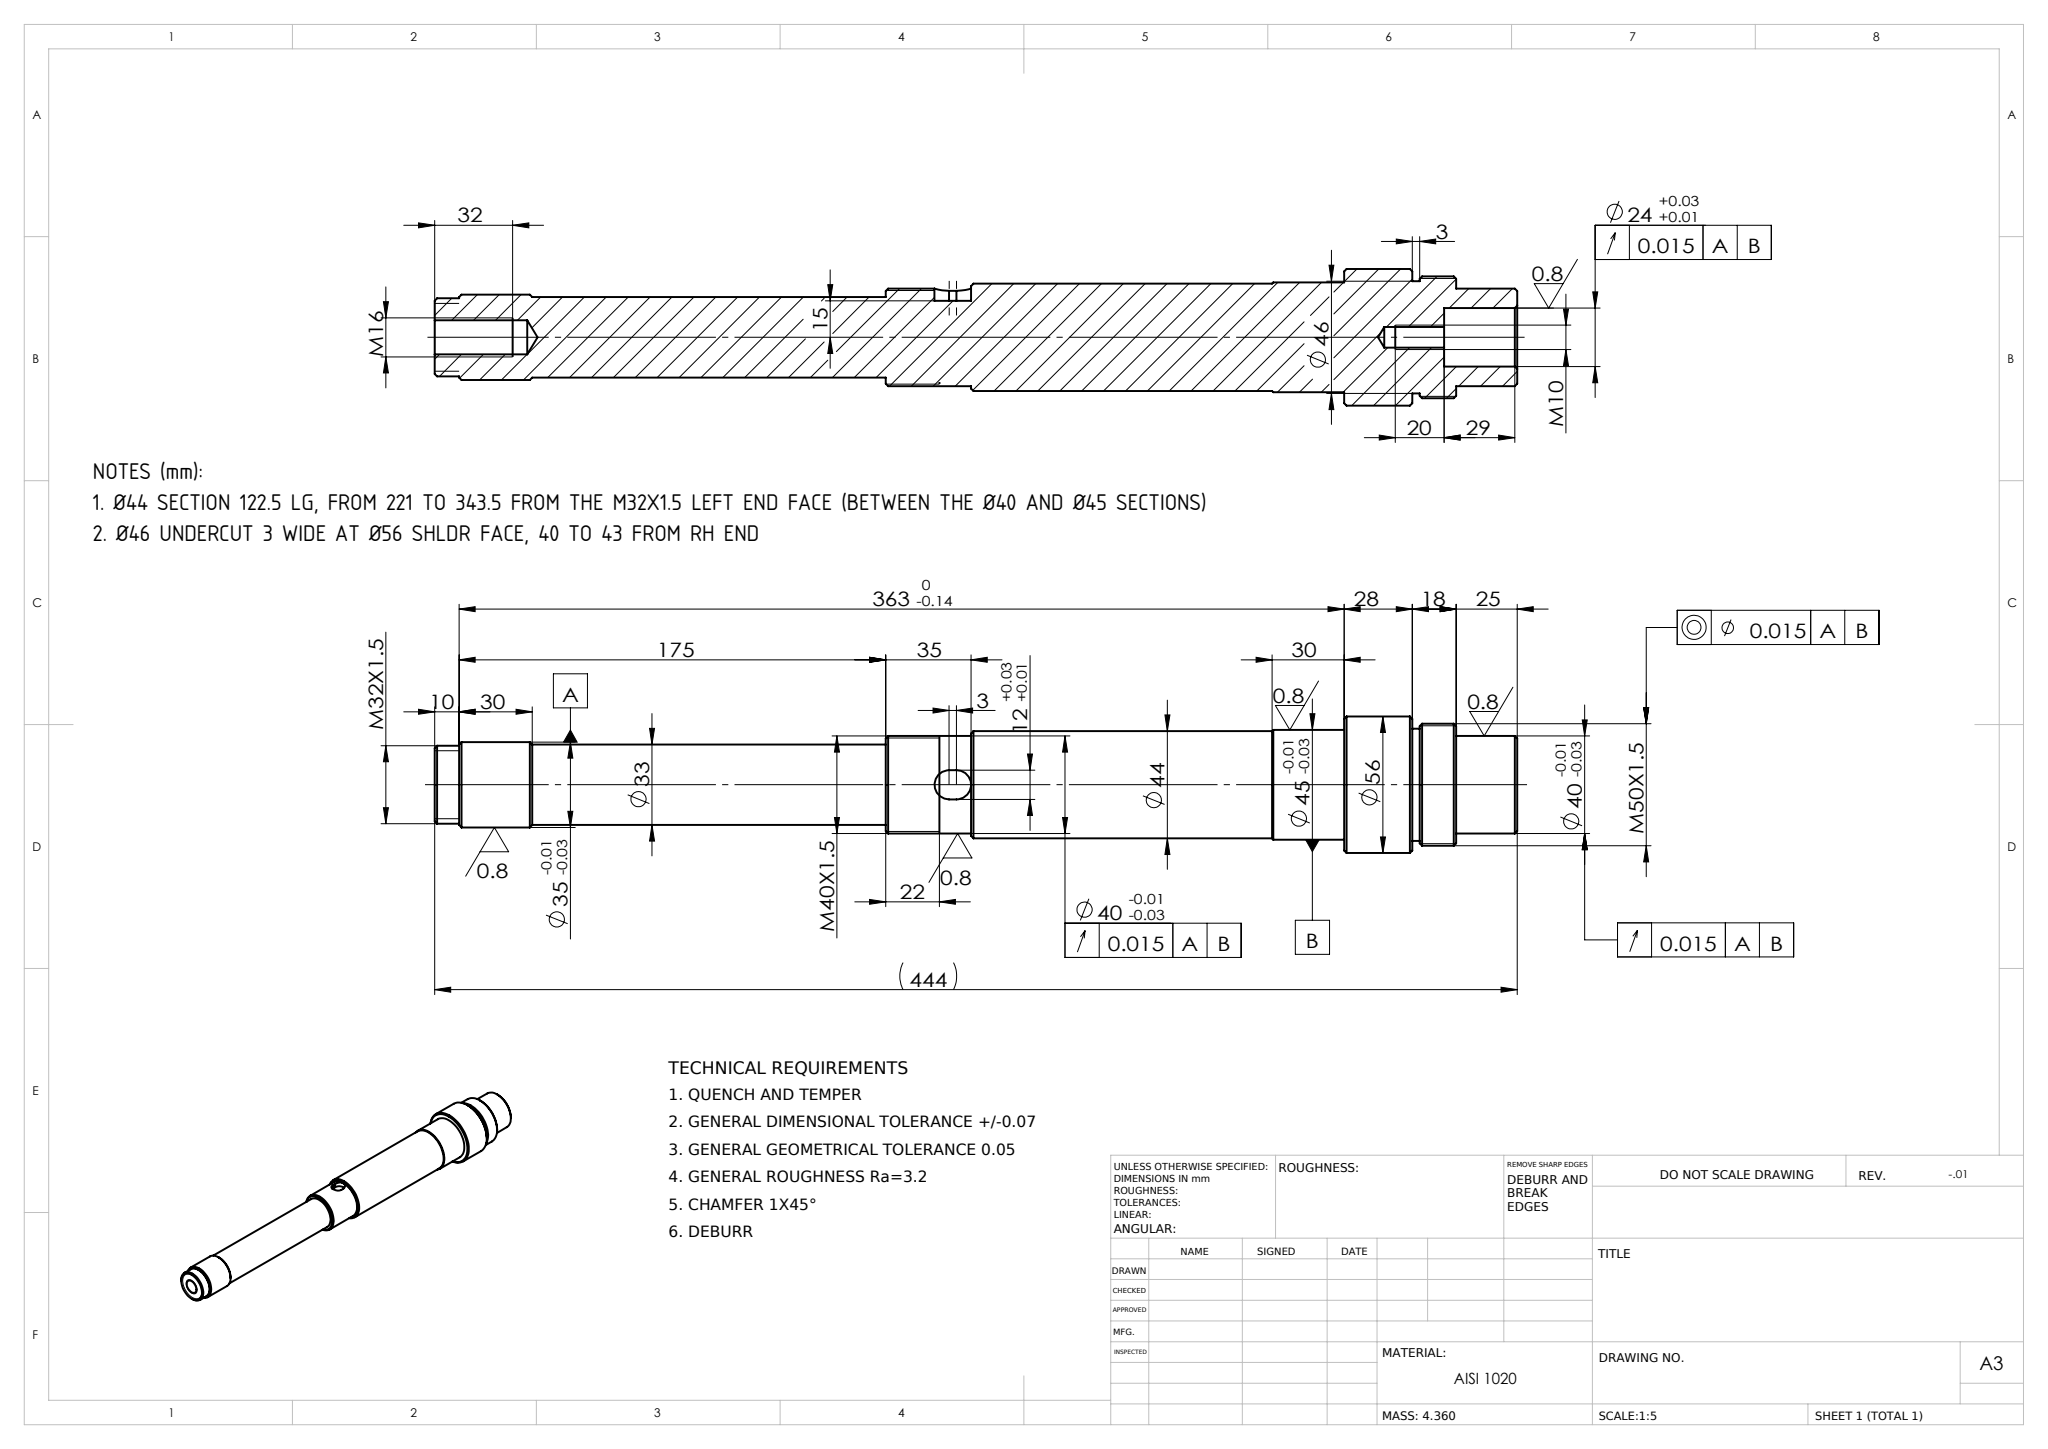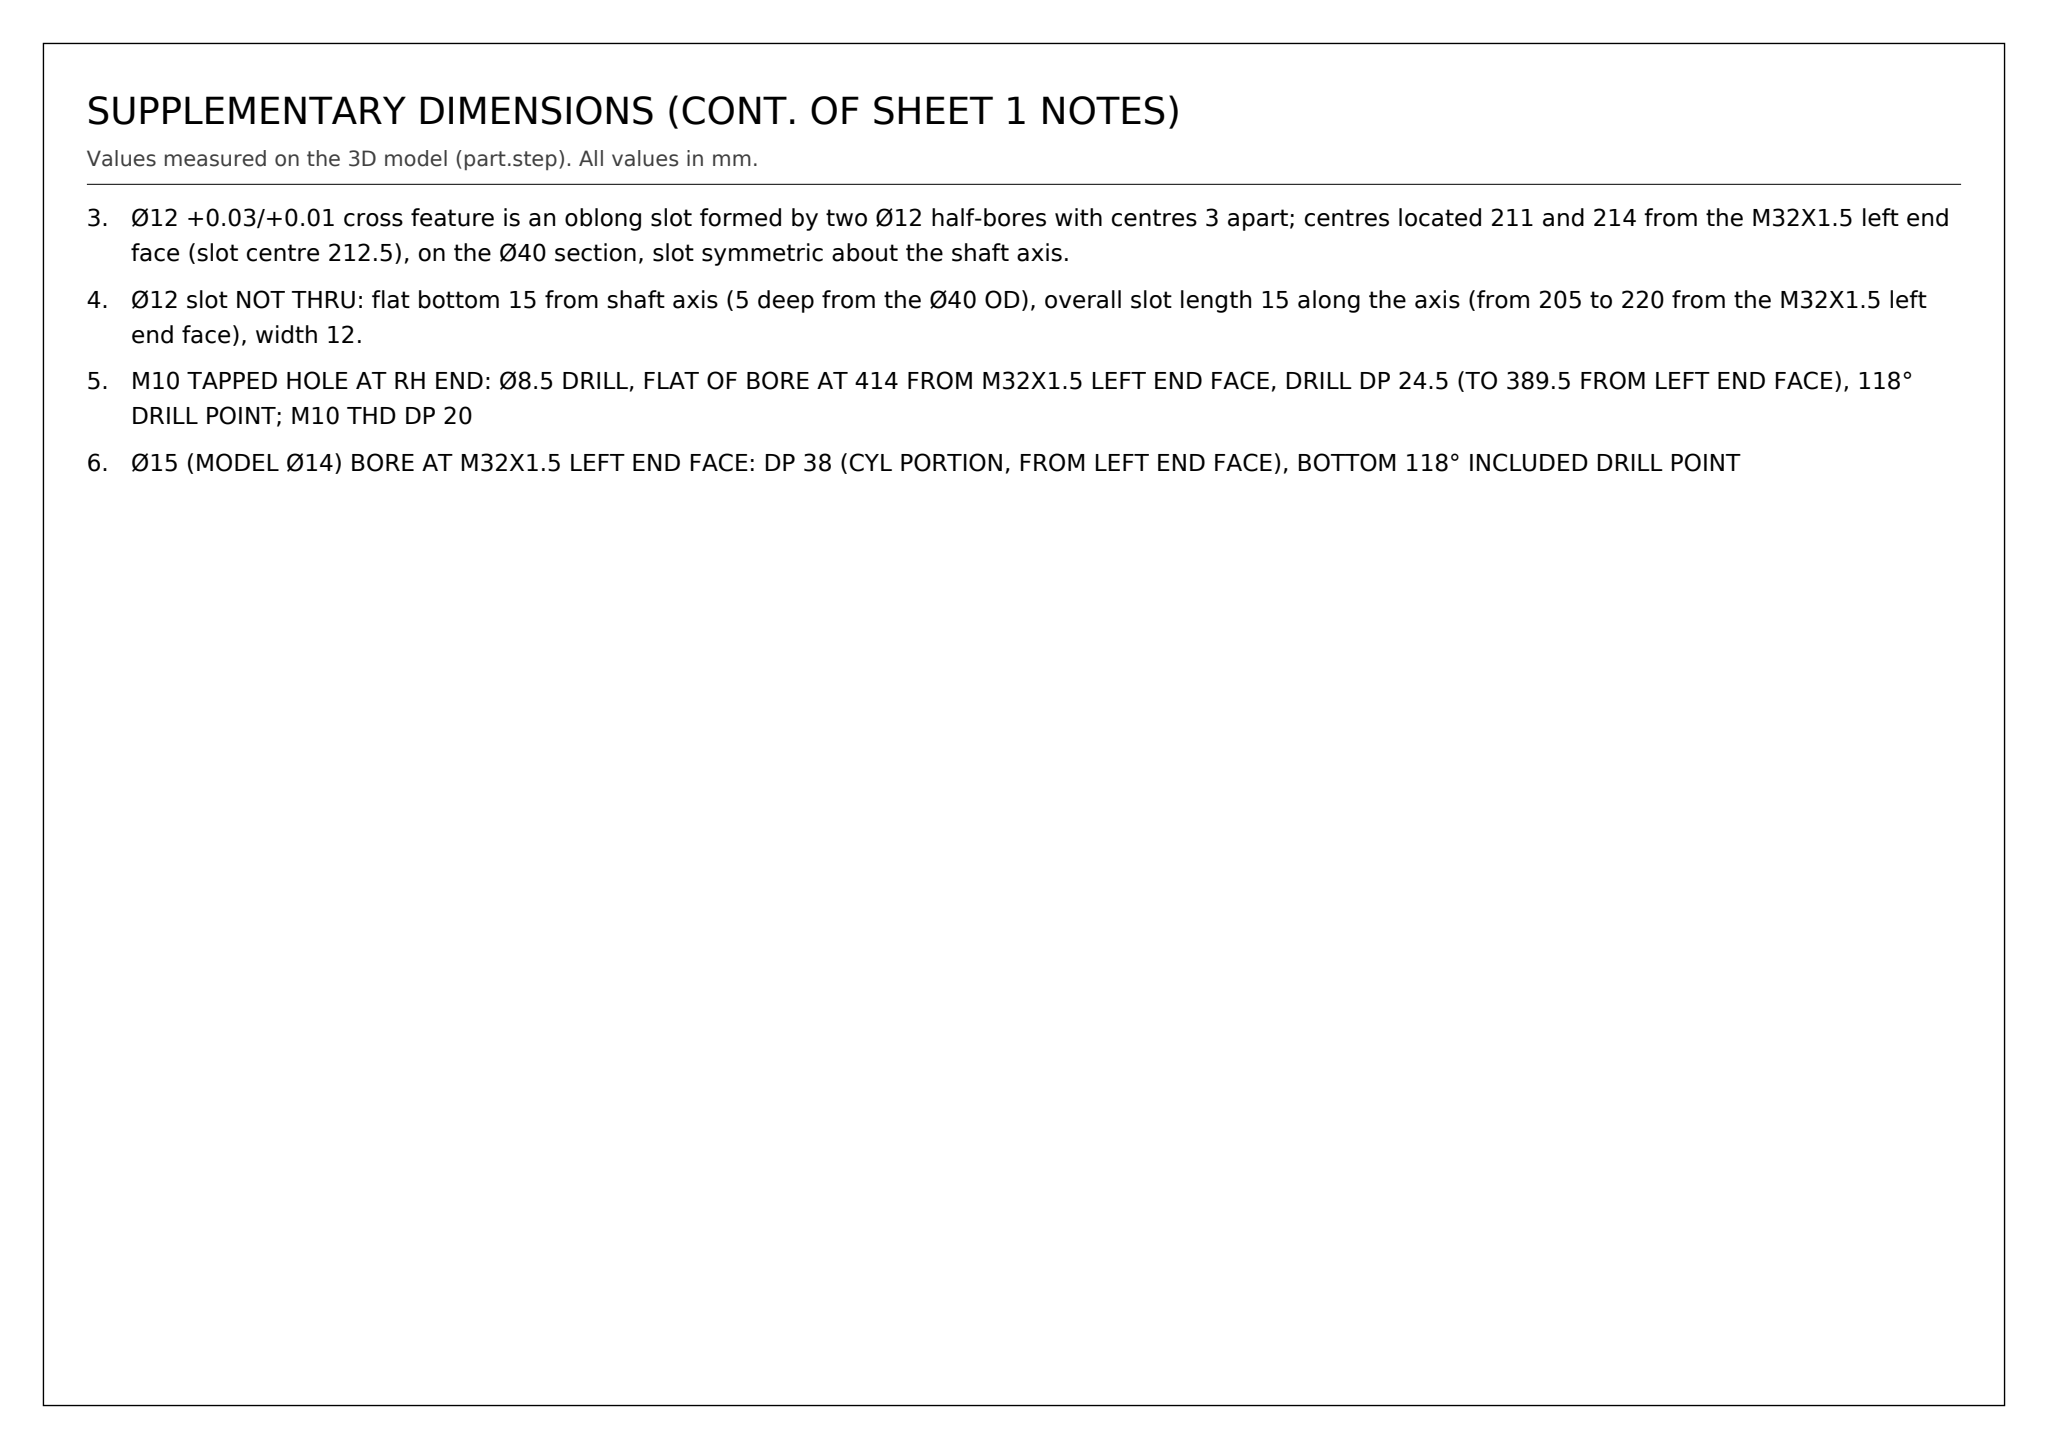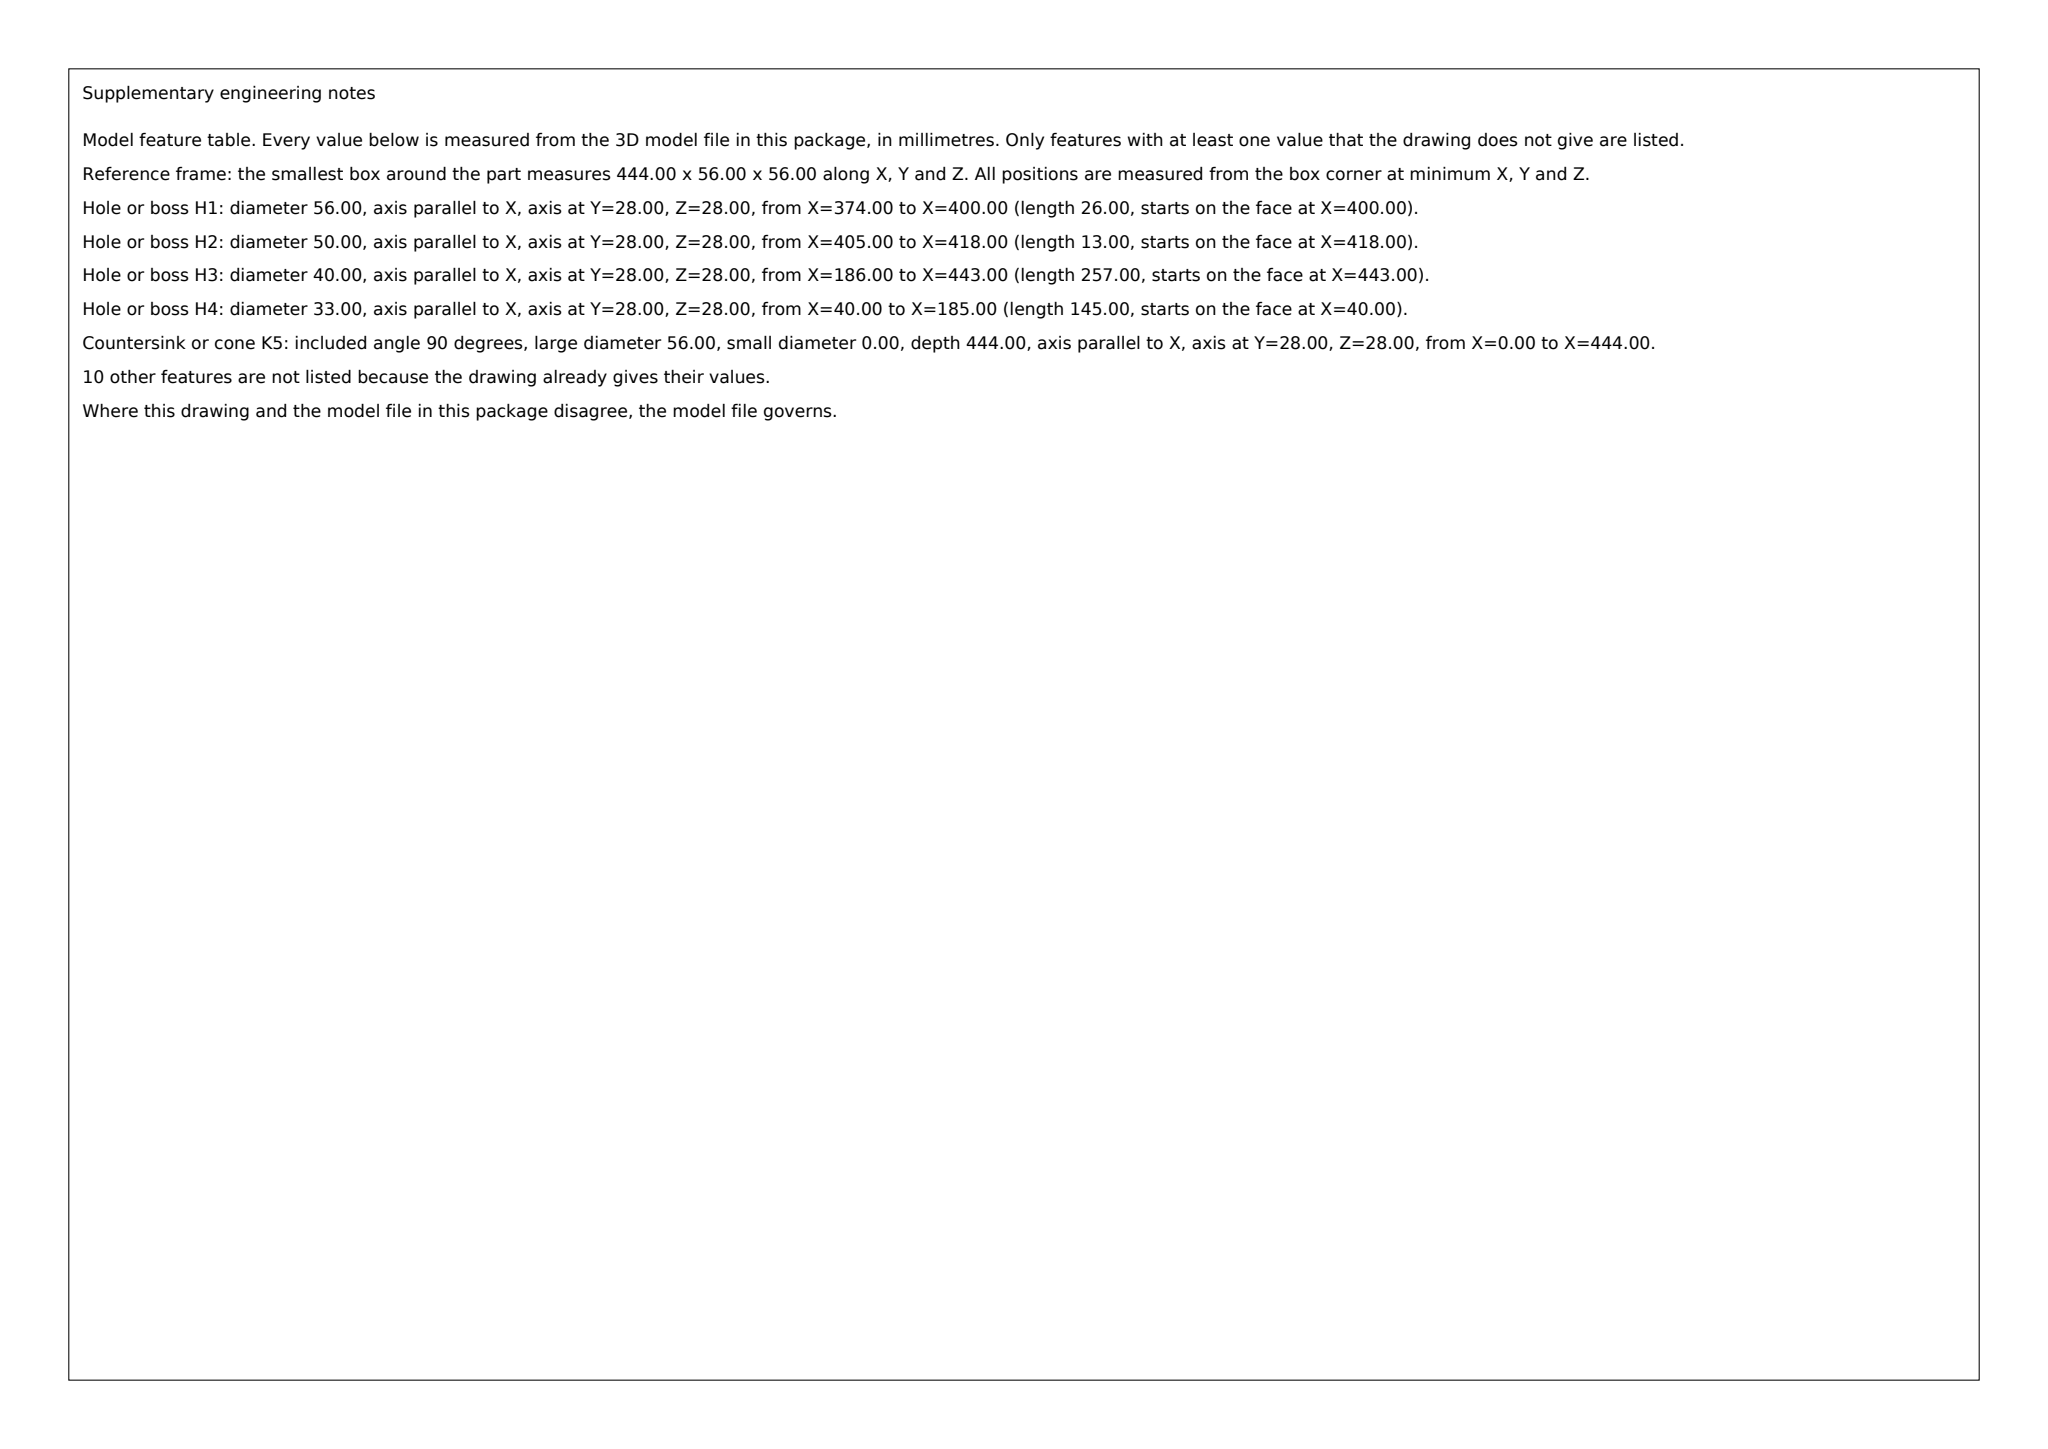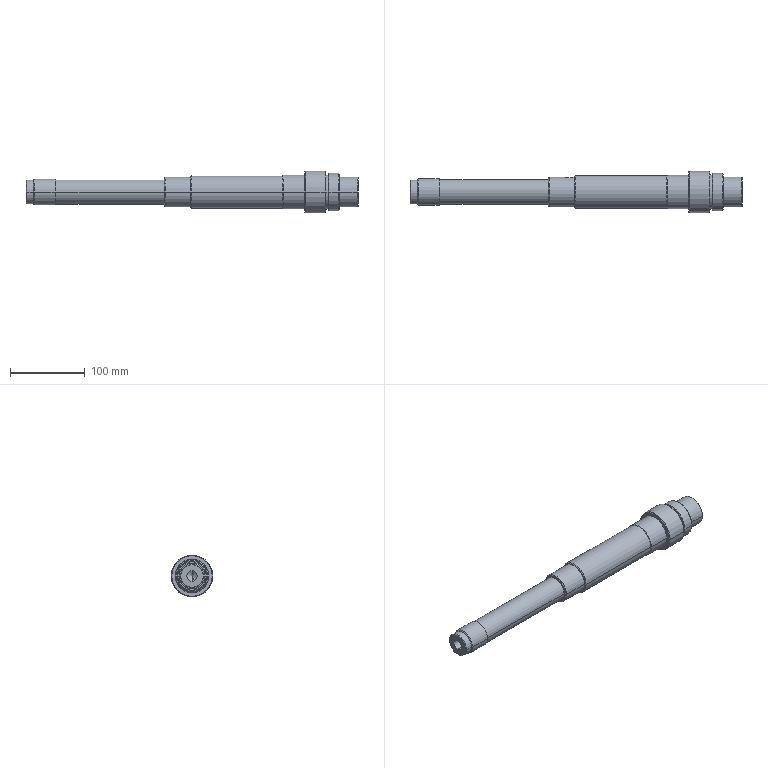Part | SolidWorks | mm | 1 solid | 70 faces | box 444 x 56 x 56 mm | volume 551910 mm3 | cylinder 29 | cone 28 | plane 13 | commonest cylinder face diameters 40 x4 12 x3 14 x2 8.5 x2 24 x2 32 x2 35 x2 33 x2
Drawing notes:
Ø44 SECTION 122.5 LG, FROM 221 TO 343.5 FROM THE M32X1.5 LEFT END FACE (BETWEEN THE Ø40 AND Ø45 SECTIONS) | from the solid: cylinders: ["boss/shaft", 44.0, "x", from 221.0 to 343.5] with adjacent ["boss/shaft", 40.0, "x", from 186.0 to 220.0] and ["boss/shaft", 45.0, "x", from 344.0 to 373.0]
Ø46 UNDERCUT 3 WIDE AT Ø56 SHLDR FACE, 40 TO 43 FROM RH END | from the solid: Cylinder dia 46, axis x, length 3 between x=401 and x=404; RH end face x=444
Ø12 +0.03/+0.01 cross feature is an oblong slot formed by two Ø12 half-bores with centres 3 apart; centres located 211 and 214 from the M32X1.5 left end face (slot centre 212.5), on the Ø40 section, slot symmetric about the shaft axis. | from the solid: cylinders: two concave arcs dia 12.0, axis y, at x=211.0 and x=214.0, z=28.0 (shaft axis y=z=28)
Ø12 slot NOT THRU: flat bottom 15 from shaft axis (5 deep from the Ø40 OD), overall slot length 15 along the axis (from 205 to 220 from the M32X1.5 left end face), width 12. | from the solid: axis plane y=43 extent x[205,220] z[22,34] (bottom face); Ø12 arcs span y 43.0 to 48.0 = Ø40 OD surface
M10 TAPPED HOLE AT RH END: Ø8.5 DRILL, FLAT OF BORE AT 414 FROM M32X1.5 LEFT END FACE, DRILL DP 24.5 (TO 389.5 FROM LEFT END FACE), 118° DRILL POINT; M10 THD DP 20 | from the solid: cylinders: hole/bore Ø8.5 on x axis from 389.5 to 414; cones 118° ref_dia 8.5 at bbox_from x=386.9; hole/bore Ø24 from 414 to 443
Ø15 (MODEL Ø14) BORE AT M32X1.5 LEFT END FACE: DP 38 (CYL PORTION, FROM LEFT END FACE), BOTTOM 118° INCLUDED DRILL POINT | from the solid: cones: [118.0 included angle, ref_dia 14.0, bbox_from x=38.0] with cylinders hole/bore Ø14.0 on x axis from 0.0 to 38.0